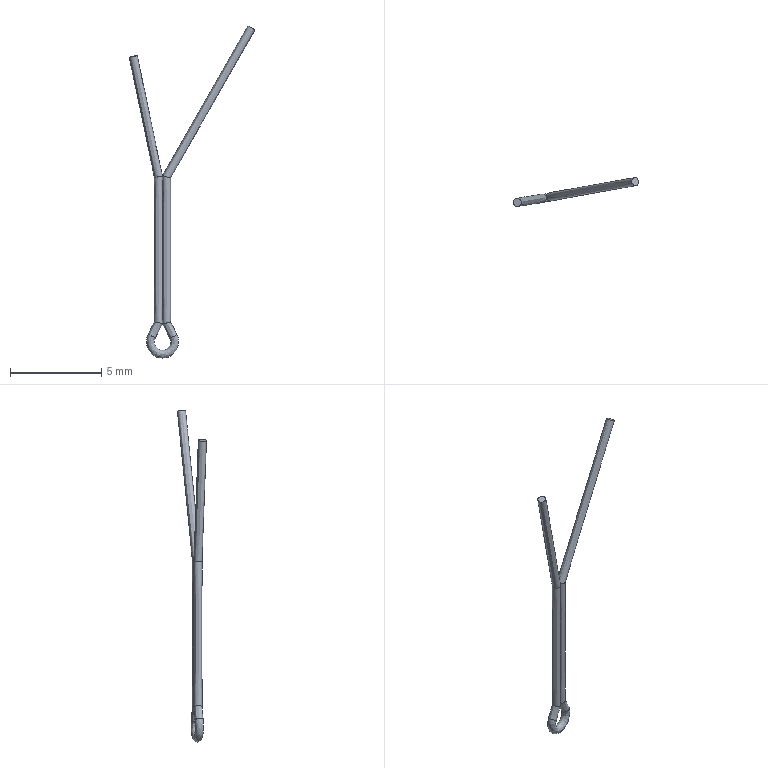Component | NX | PIN | 1 solid | 9 faces | volume 6 mm3 | spline 7 | plane 2